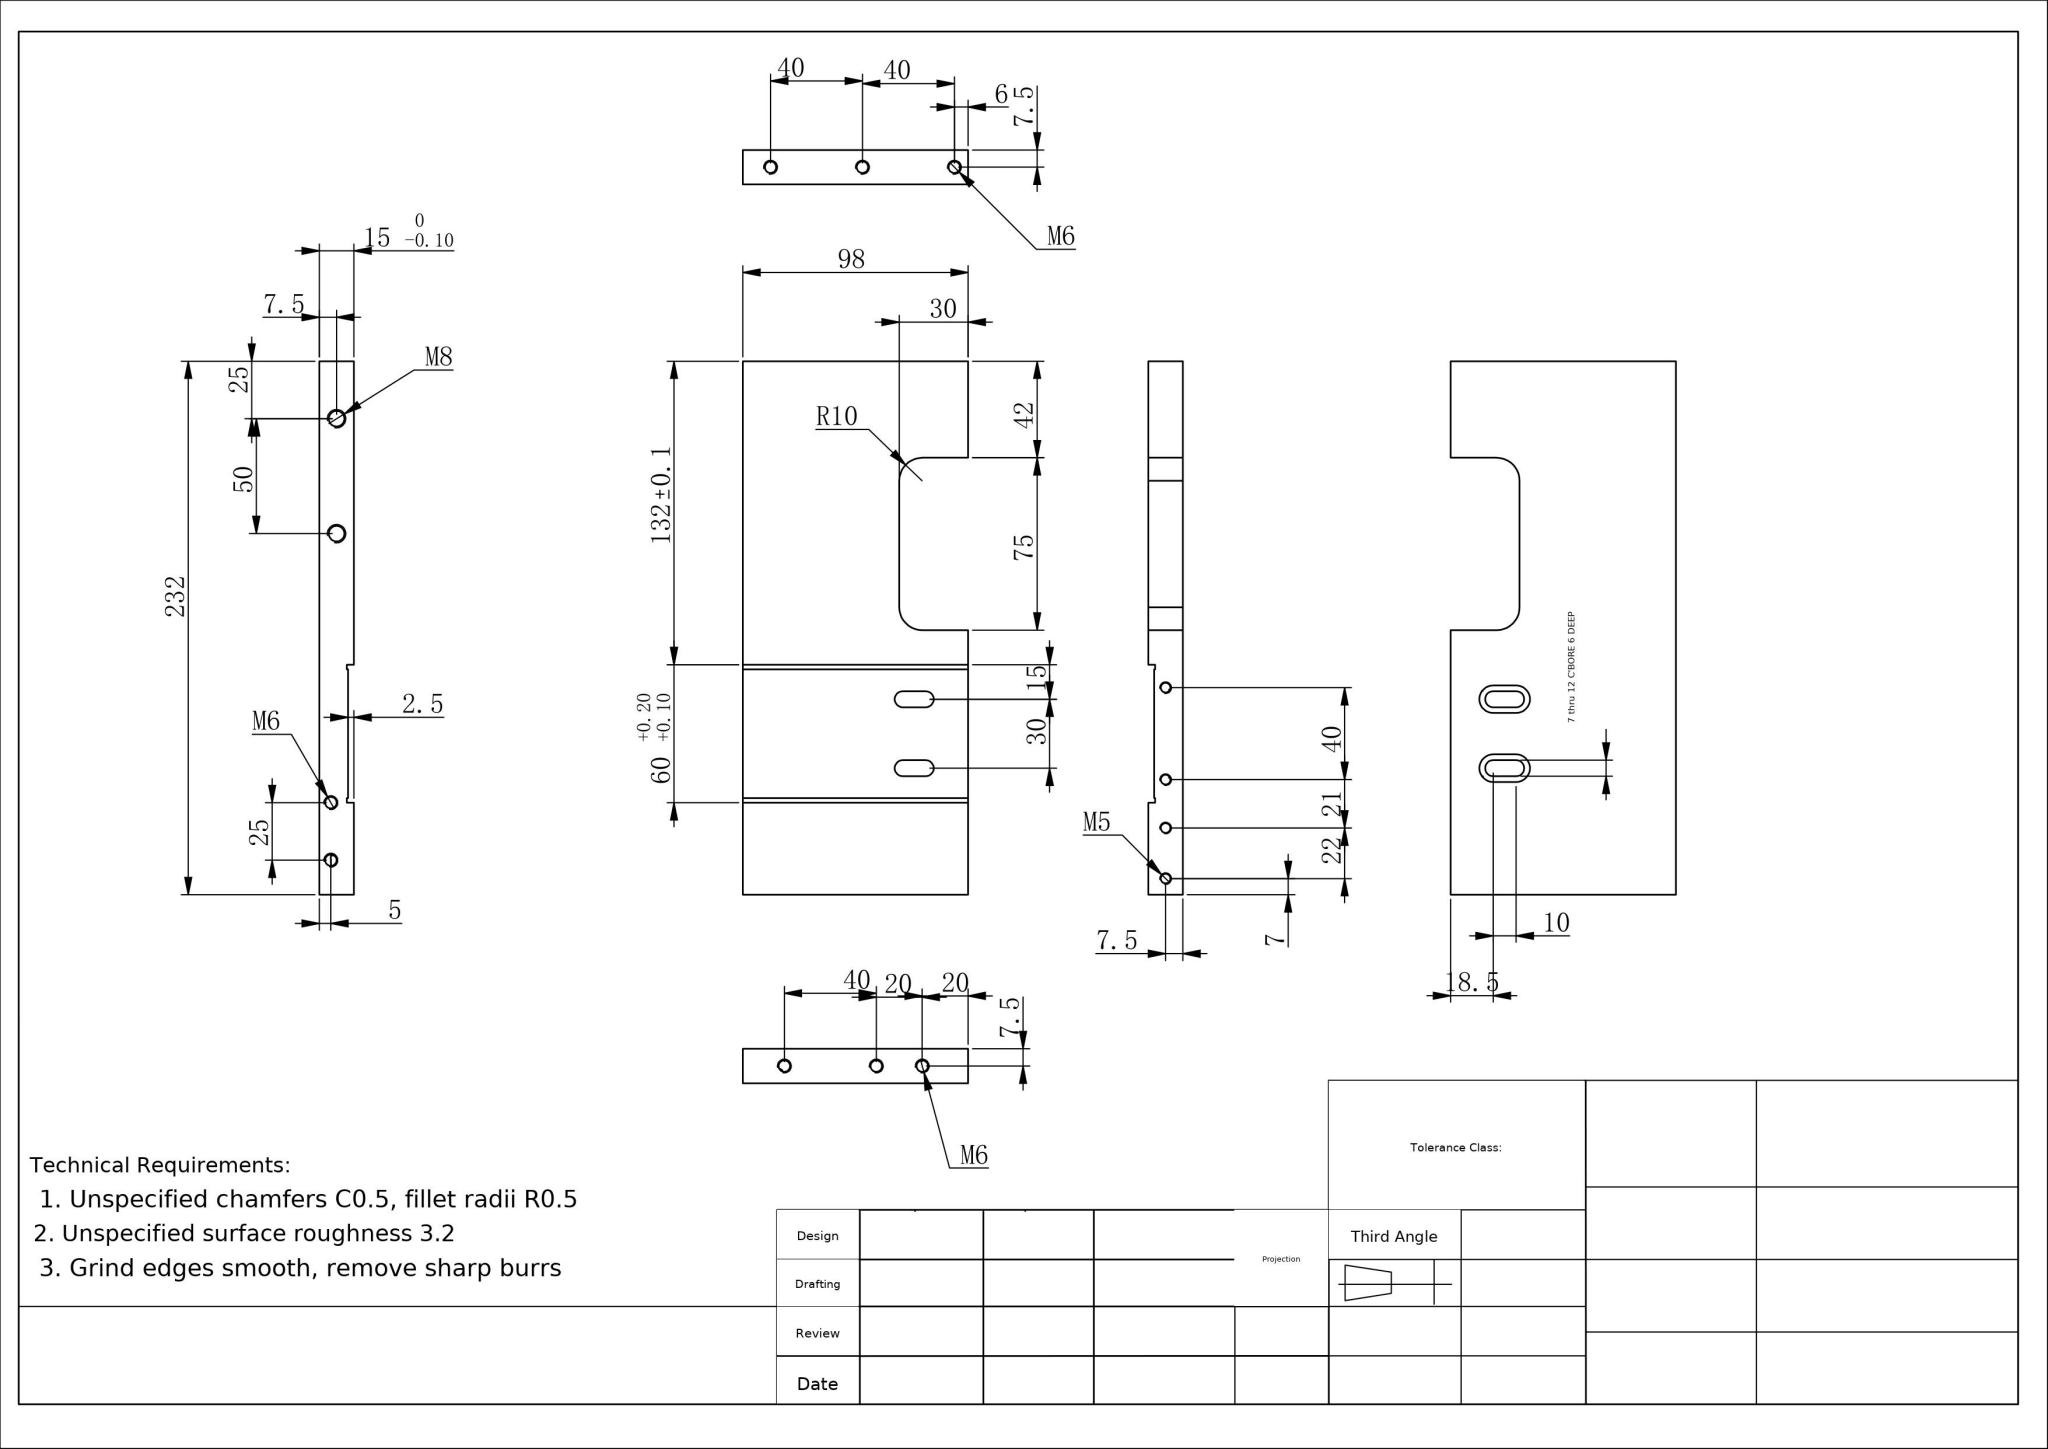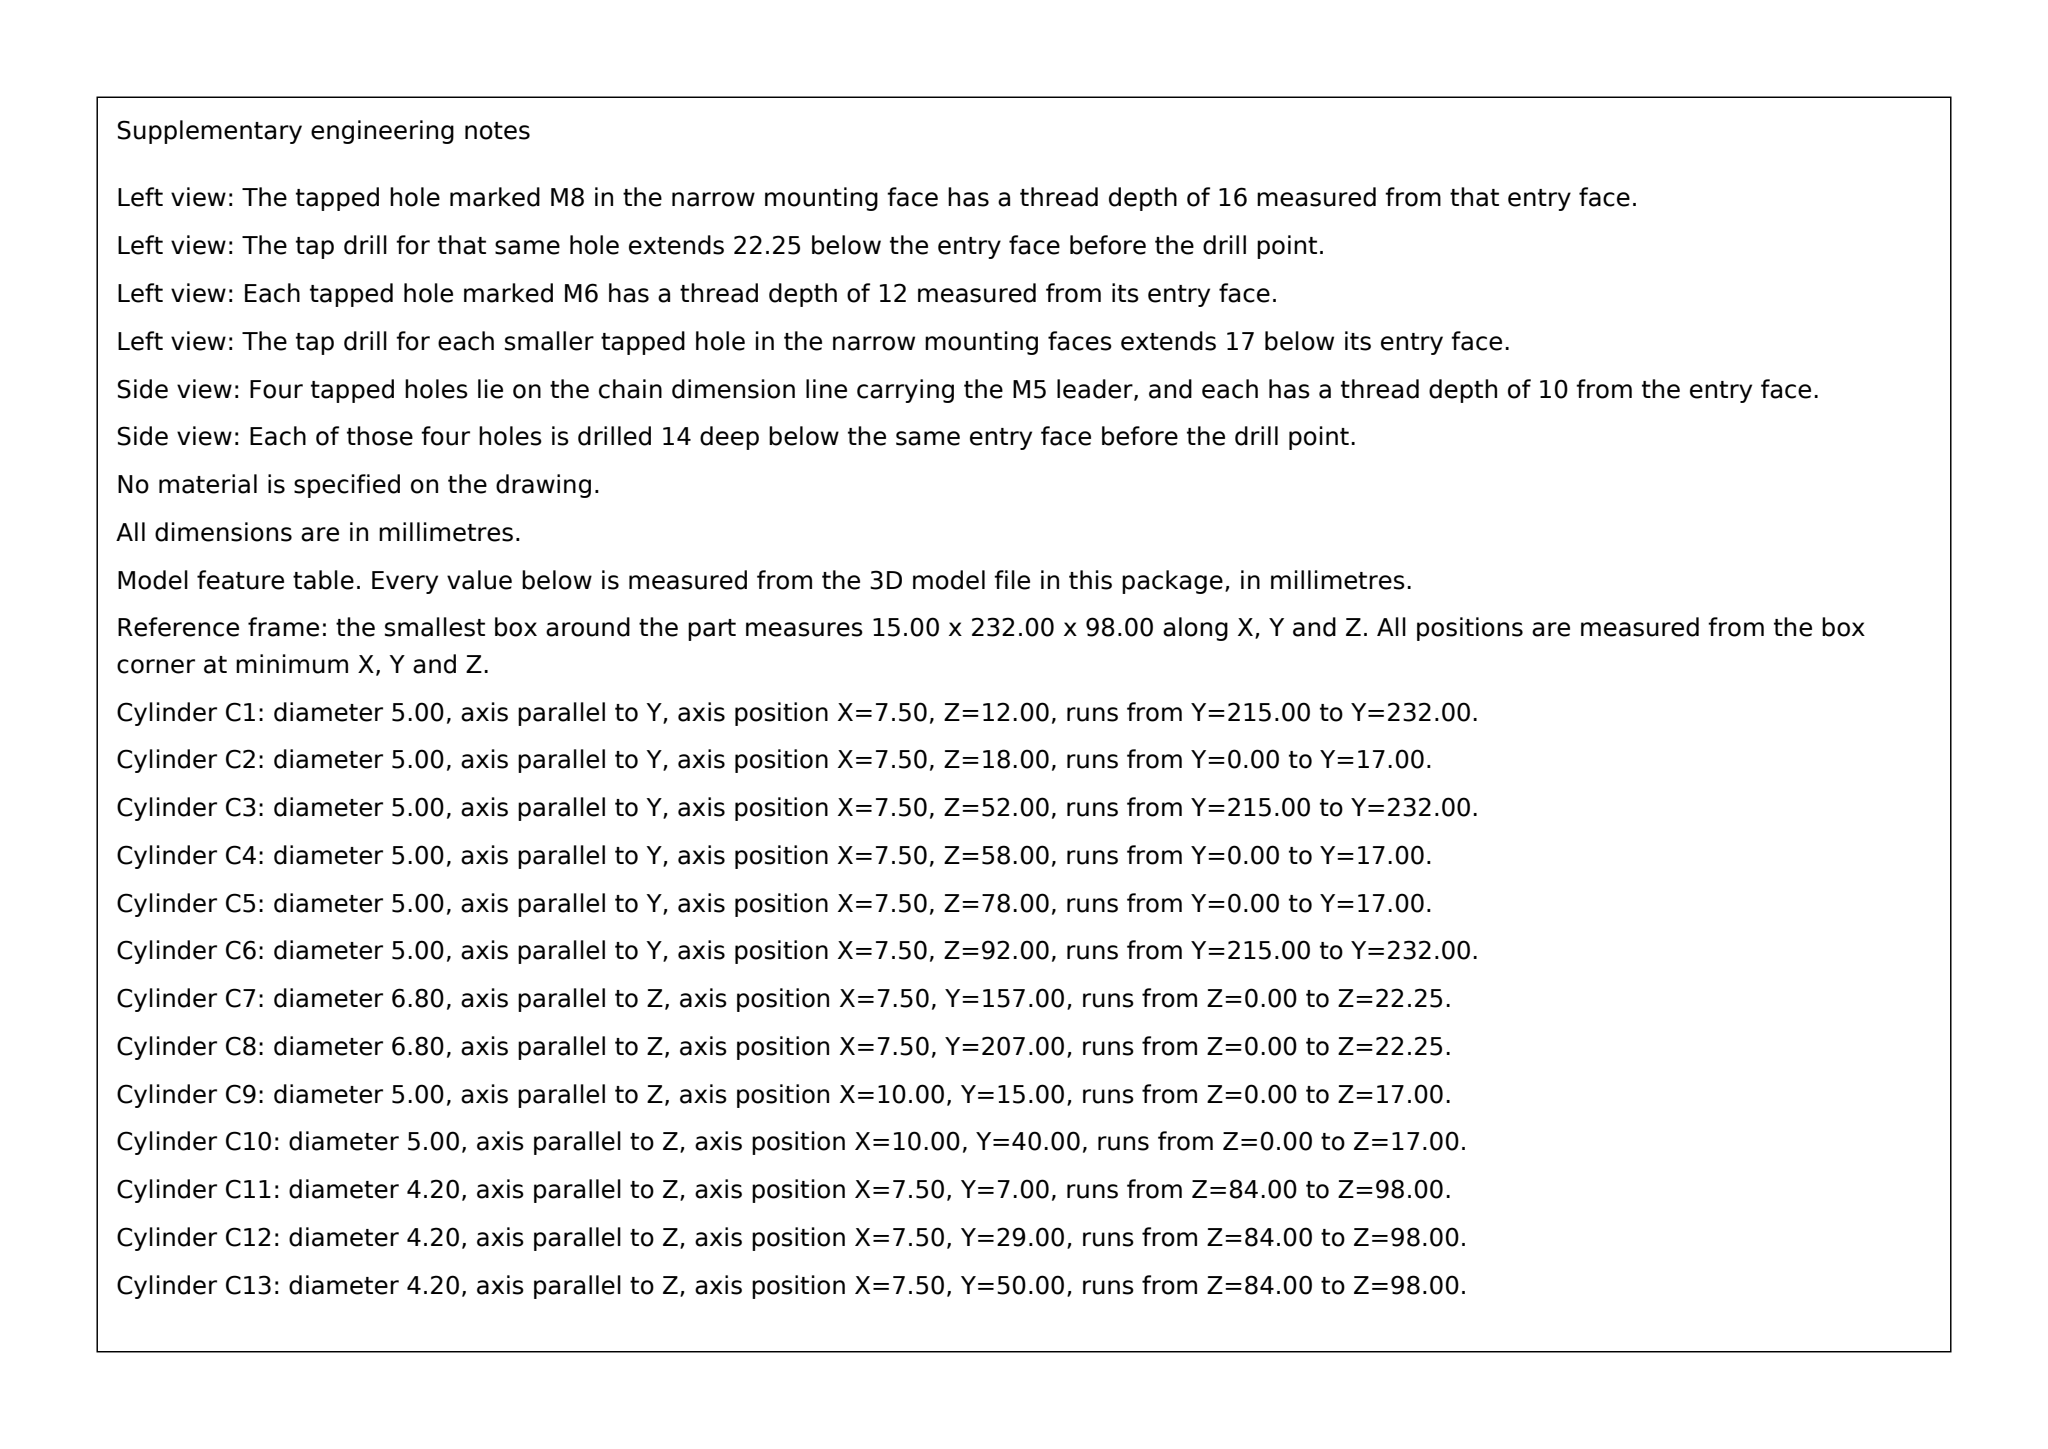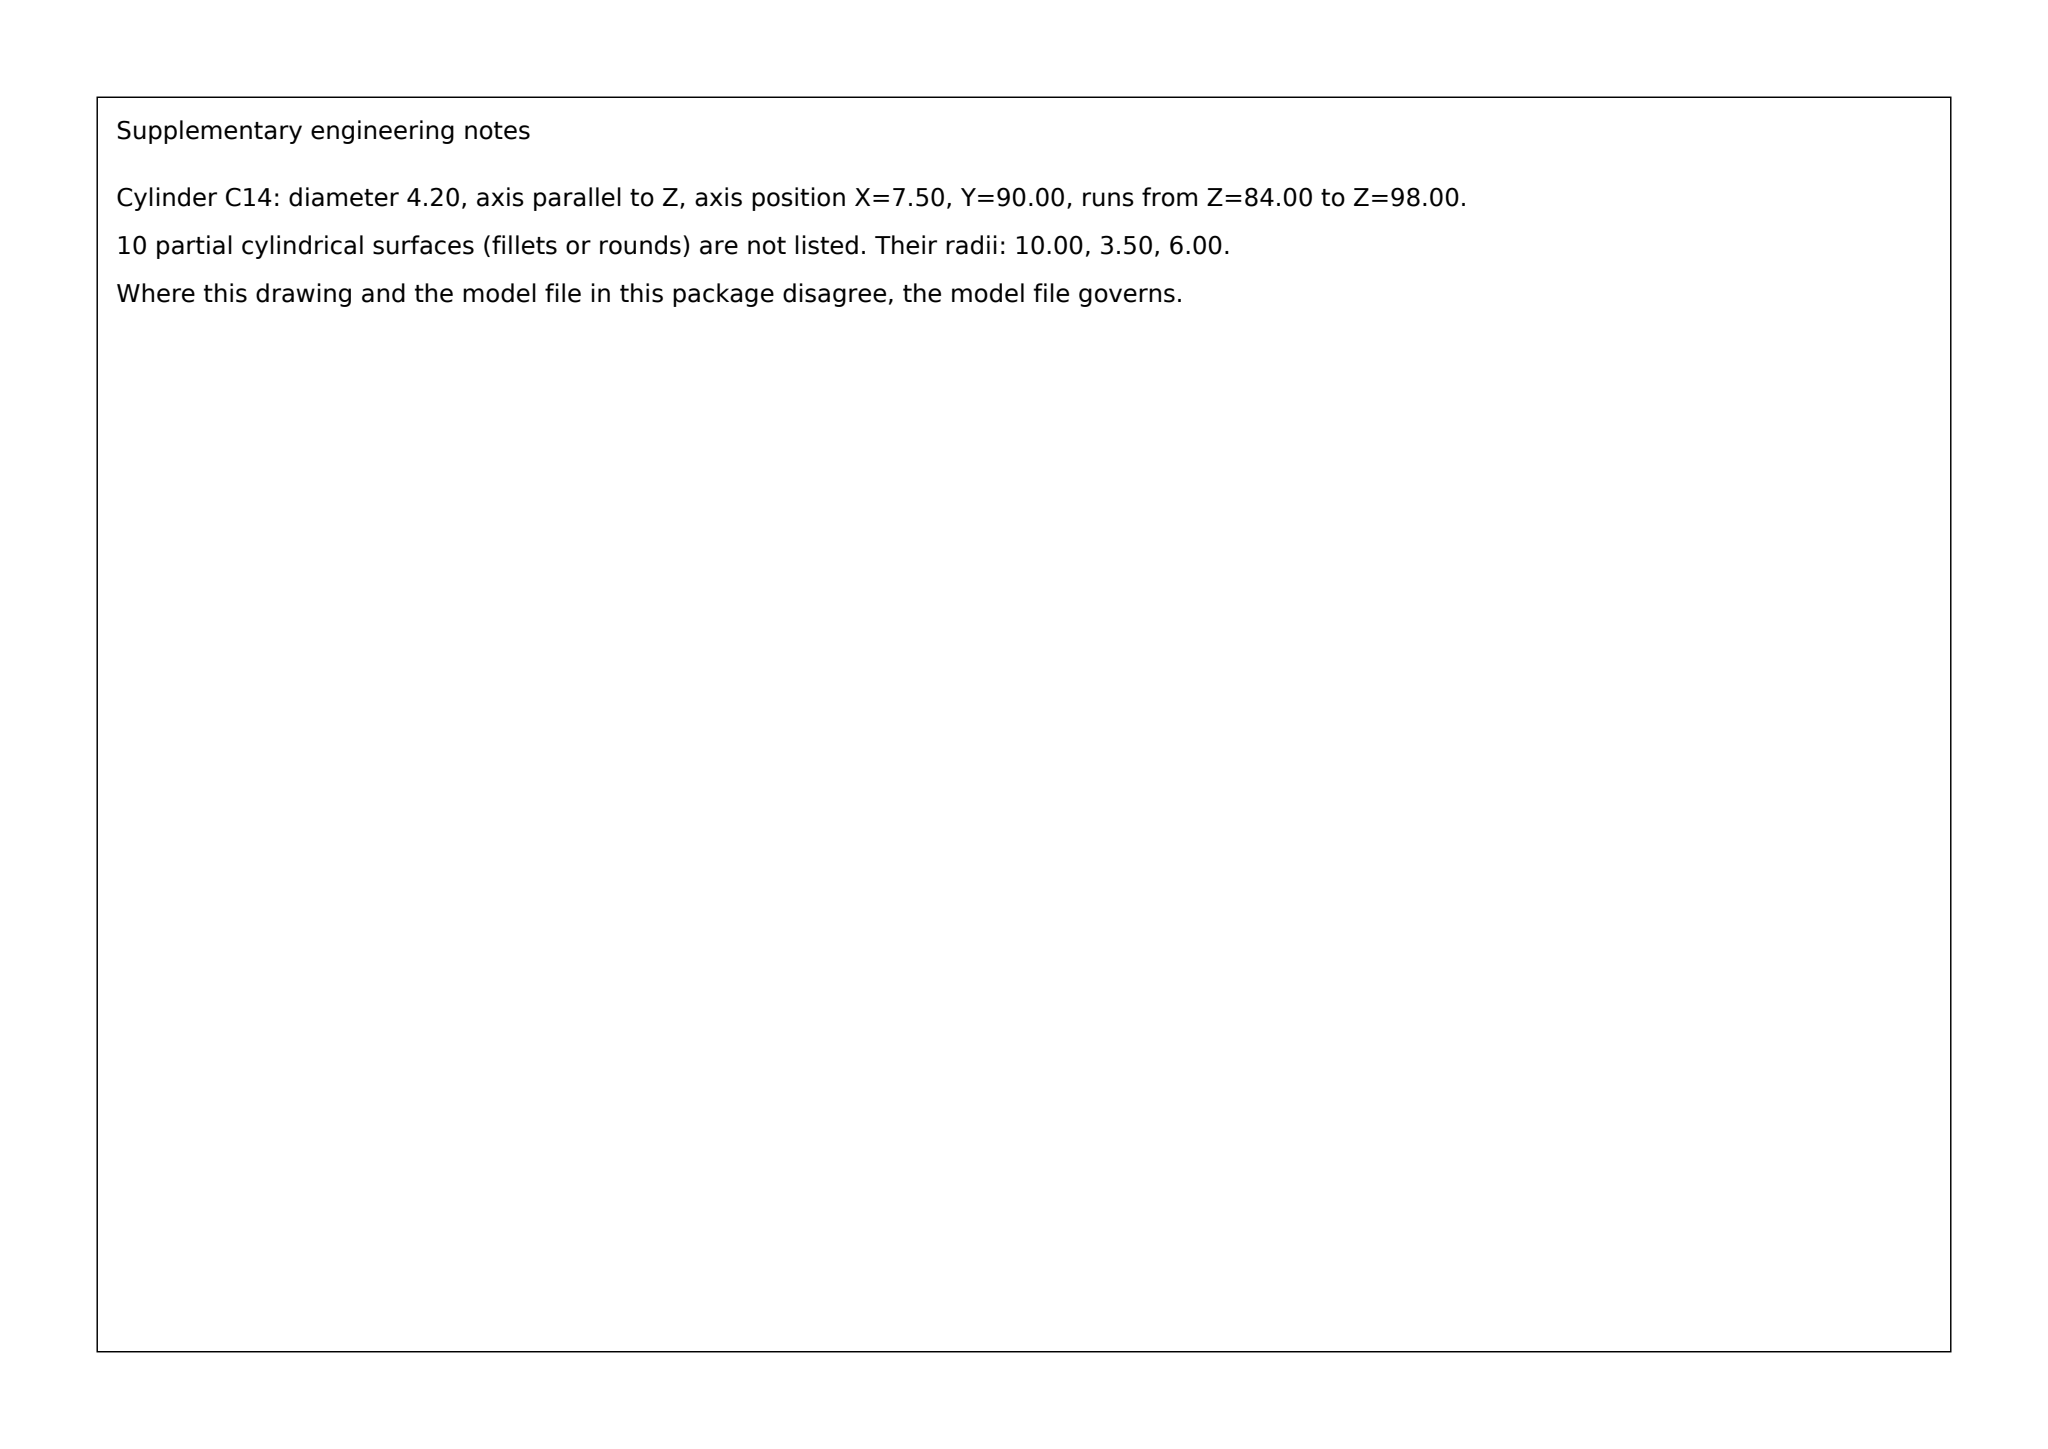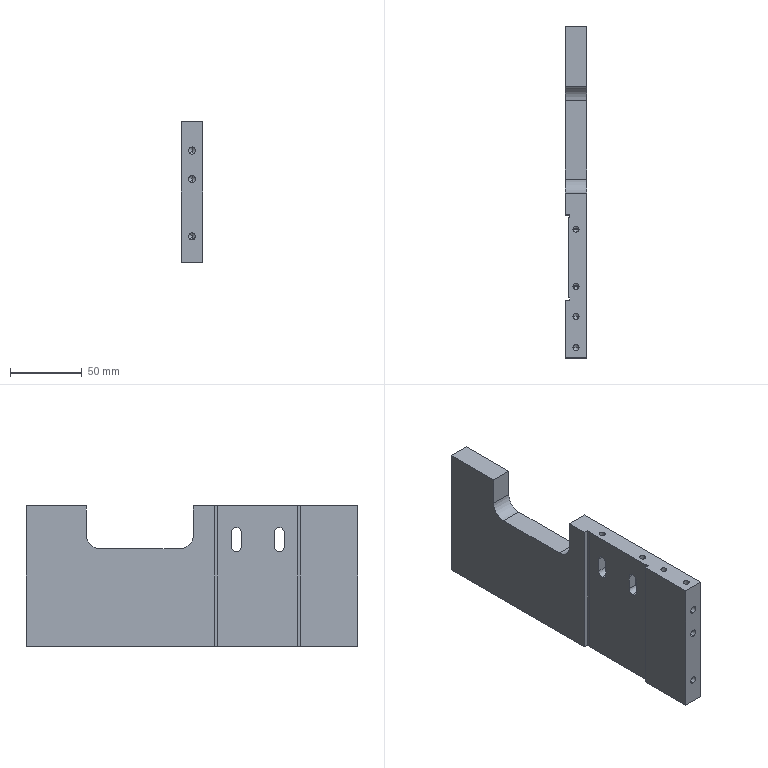Part | SolidWorks | mm | 1 solid | 99 faces | box 15 x 232 x 98 mm | volume 283630 mm3 | cylinder 43 | cone 28 | plane 28 | commonest cylinder face diameters 5 x17 4.2 x8 12 x6 7 x6 6.8 x4 20 x2
Drawing notes:
SIDE VIEW STEPS: 6 DEEP TO FACE @9, 12 DEEP TO FACE @3 FR 15 FACE | from the solid: axis_planes x = 0, 2.5, 3.0, 9.0, 15.0 over 15 THK
2 WIDE LEDGES AT STEPS: Y 40-42 & 98-100 FROM BOT END | from the solid: axis_planes y = 40, 42, 98, 100
STEPPED BAND 60 LG: 40 FROM BOT END, 132 FROM TOP END, 232 OAL | from the solid: y planes 40 & 100 within 232 bbox length
LOWER 2X M6 DP 17: 15 FROM BOT EDGE TO 1ST HOLE, 25 PITCH | from the solid: Ø5 z-axis holes at y = 15.0 and y = 40.0
2X M6 DP 17 CL 10 FROM BACK FACE (5 FROM OPP FACE, 15 THK) | from the solid: Ø5 z-axis holes at x = 10.0 in 15 THK
build123d program:
from build123d import *

# Parameters (mm, degrees)
SKETCH1_W             = 98
SKETCH1_H             = 232
BOSS_EXTRUDE1_DEPTH   = 15
CUT_EXTRUDE1_DEPTH    = 253.295
SKETCH3_W             = 2.5
SKETCH3_H             = 60
CUT_EXTRUDE2_DEPTH    = 120
SKETCH4_W             = 98
SKETCH4_H             = 2
CUT_EXTRUDE3_DEPTH    = 0.5
M6_TAPPED_HOLE1_D     = 5
M6_TAPPED_HOLE1_DEPTH = 17
M6_TAPPED_HOLE1_TIP   = 1.502
M5_TAPPED_HOLE1_D     = 4.2
M5_TAPPED_HOLE1_DEPTH = 14
M5_TAPPED_HOLE1_TIP   = 1.262
M5_TAPPED_HOLE2_D     = 4.2
M5_TAPPED_HOLE2_DEPTH = 14
M5_TAPPED_HOLE2_TIP   = 1.262
M6_TAPPED_HOLE2_D     = 5
M6_TAPPED_HOLE2_DEPTH = 17
M6_TAPPED_HOLE2_TIP   = 1.502
M6_TAPPED_HOLE3_D     = 5
M6_TAPPED_HOLE3_DEPTH = 17
M6_TAPPED_HOLE3_TIP   = 1.502
CUT_EXTRUDE4_DEPTH    = 253.295
CUT_EXTRUDE5_DEPTH    = 6
M8_TAPPED_HOLE2_D     = 6.8
M8_TAPPED_HOLE2_DEPTH = 22.25
M8_TAPPED_HOLE2_TIP   = 2.043


with BuildPart() as part:
    # Sketch1 → Boss-Extrude1 (new body)
    with BuildSketch(Plane(origin=(0, 0, 0), x_dir=(0, 0, -1), z_dir=(1, 0, 0))):
        with Locations((49, 116)):
            Rectangle(SKETCH1_W, SKETCH1_H)
    extrude(amount=BOSS_EXTRUDE1_DEPTH)

    # Sketch2 → Cut-Extrude1 (cut, through all)
    with BuildSketch(Plane.ZY):
        with BuildLine():
            Line((0, 115), (-20, 115))
            ThreePointArc((-20, 115), (-27.071, 117.929), (-30, 125))
            Line((-30, 125), (-30, 180))
            ThreePointArc((-30, 180), (-27.071, 187.071), (-20, 190))
            Line((-20, 190), (0, 190))
            Line((0, 190), (0, 115))
        make_face()
    extrude(amount=-CUT_EXTRUDE1_DEPTH, mode=Mode.SUBTRACT)

    # Sketch3 → Cut-Extrude2 (cut)
    with BuildSketch(Plane.XY):
        with Locations((1.25, 70)):
            Rectangle(SKETCH3_W, SKETCH3_H)
    extrude(amount=-CUT_EXTRUDE2_DEPTH, mode=Mode.SUBTRACT)

    # Sketch4 → Cut-Extrude3 (cut)
    with BuildSketch(Plane.ZY.offset(-2.5)):
        with Locations((-49, 99)):
            Rectangle(SKETCH4_W, SKETCH4_H)
        with Locations((-49, 41)):
            Rectangle(SKETCH4_W, SKETCH4_H)
    extrude(amount=-CUT_EXTRUDE3_DEPTH, mode=Mode.SUBTRACT)

    # M6 Tapped Hole1
    with Locations(Plane(origin=(0, 232, 0), x_dir=(1, 0, 0), z_dir=(0, 1, 0))):
        with Locations((7.5, 86), (7.5, 46), (7.5, 6)):
            Hole(M6_TAPPED_HOLE1_D / 2, depth=M6_TAPPED_HOLE1_DEPTH)
            with Locations((0, 0, -(M6_TAPPED_HOLE1_DEPTH + M6_TAPPED_HOLE1_TIP / 2))):  # 118° drill point
                Cone(0, M6_TAPPED_HOLE1_D / 2, M6_TAPPED_HOLE1_TIP, mode=Mode.SUBTRACT)

    # M5 Tapped Hole1
    with Locations(Plane.XY):
        with Locations((7.5, 90), (7.5, 50)):
            Hole(M5_TAPPED_HOLE1_D / 2, depth=M5_TAPPED_HOLE1_DEPTH)
            with Locations((0, 0, -(M5_TAPPED_HOLE1_DEPTH + M5_TAPPED_HOLE1_TIP / 2))):  # 118° drill point
                Cone(0, M5_TAPPED_HOLE1_D / 2, M5_TAPPED_HOLE1_TIP, mode=Mode.SUBTRACT)

    # M5 Tapped Hole2
    with Locations(Plane.XY):
        with Locations((7.5, 29), (7.5, 7)):
            Hole(M5_TAPPED_HOLE2_D / 2, depth=M5_TAPPED_HOLE2_DEPTH)
            with Locations((0, 0, -(M5_TAPPED_HOLE2_DEPTH + M5_TAPPED_HOLE2_TIP / 2))):  # 118° drill point
                Cone(0, M5_TAPPED_HOLE2_D / 2, M5_TAPPED_HOLE2_TIP, mode=Mode.SUBTRACT)

    # M6 Tapped Hole2
    with Locations(Plane(origin=(0, 0, 0), x_dir=(-1, 0, 0), z_dir=(0, -1, 0))):
        with Locations((-7.5, 20), (-7.5, 40), (-7.5, 80)):
            Hole(M6_TAPPED_HOLE2_D / 2, depth=M6_TAPPED_HOLE2_DEPTH)
            with Locations((0, 0, -(M6_TAPPED_HOLE2_DEPTH + M6_TAPPED_HOLE2_TIP / 2))):  # 118° drill point
                Cone(0, M6_TAPPED_HOLE2_D / 2, M6_TAPPED_HOLE2_TIP, mode=Mode.SUBTRACT)

    # M6 Tapped Hole3
    with Locations(Plane(origin=(0, 0, -98), x_dir=(-1, 0, 0), z_dir=(0, 0, -1))):
        with Locations((-10, 15), (-10, 40)):
            Hole(M6_TAPPED_HOLE3_D / 2, depth=M6_TAPPED_HOLE3_DEPTH)
            with Locations((0, 0, -(M6_TAPPED_HOLE3_DEPTH + M6_TAPPED_HOLE3_TIP / 2))):  # 118° drill point
                Cone(0, M6_TAPPED_HOLE3_D / 2, M6_TAPPED_HOLE3_TIP, mode=Mode.SUBTRACT)

    # Sketch18 → Cut-Extrude4 (cut, through all)
    with BuildSketch(Plane(origin=(15, 0, 0), x_dir=(0, 0, -1), z_dir=(1, 0, 0))):
        with BuildLine():
            Line((18.5, 58.5), (28.5, 58.5))
            ThreePointArc((28.5, 58.5), (32, 55), (28.5, 51.5))
            Line((28.5, 51.5), (18.5, 51.5))
            ThreePointArc((18.5, 51.5), (15, 55), (18.5, 58.5))
        make_face()
        with BuildLine():
            Line((28.5, 81.5), (18.5, 81.5))
            ThreePointArc((18.5, 81.5), (15, 85), (18.5, 88.5))
            Line((18.5, 88.5), (28.5, 88.5))
            ThreePointArc((28.5, 88.5), (32, 85), (28.5, 81.5))
        make_face()
    extrude(amount=-CUT_EXTRUDE4_DEPTH, mode=Mode.SUBTRACT)

    # Sketch19 → Cut-Extrude5 (cut)
    with BuildSketch(Plane(origin=(15, 0, 0), x_dir=(0, 0, -1), z_dir=(1, 0, 0))):
        with BuildLine():
            Line((28.5, 49), (18.5, 49))
            ThreePointArc((18.5, 49), (12.5, 55), (18.5, 61))
            Line((18.5, 61), (28.5, 61))
            ThreePointArc((28.5, 61), (34.5, 55), (28.5, 49))
        make_face()
        with BuildLine():
            Line((28.5, 79), (18.5, 79))
            ThreePointArc((18.5, 79), (12.5, 85), (18.5, 91))
            Line((18.5, 91), (28.5, 91))
            ThreePointArc((28.5, 91), (34.5, 85), (28.5, 79))
        make_face()
    extrude(amount=-CUT_EXTRUDE5_DEPTH, mode=Mode.SUBTRACT)

    # M8 Tapped Hole2
    with Locations(Plane(origin=(0, 0, -98), x_dir=(-1, 0, 0), z_dir=(0, 0, -1))):
        with Locations((-7.5, 157), (-7.5, 207)):
            Hole(M8_TAPPED_HOLE2_D / 2, depth=M8_TAPPED_HOLE2_DEPTH)
            with Locations((0, 0, -(M8_TAPPED_HOLE2_DEPTH + M8_TAPPED_HOLE2_TIP / 2))):  # 118° drill point
                Cone(0, M8_TAPPED_HOLE2_D / 2, M8_TAPPED_HOLE2_TIP, mode=Mode.SUBTRACT)


solid = part.part